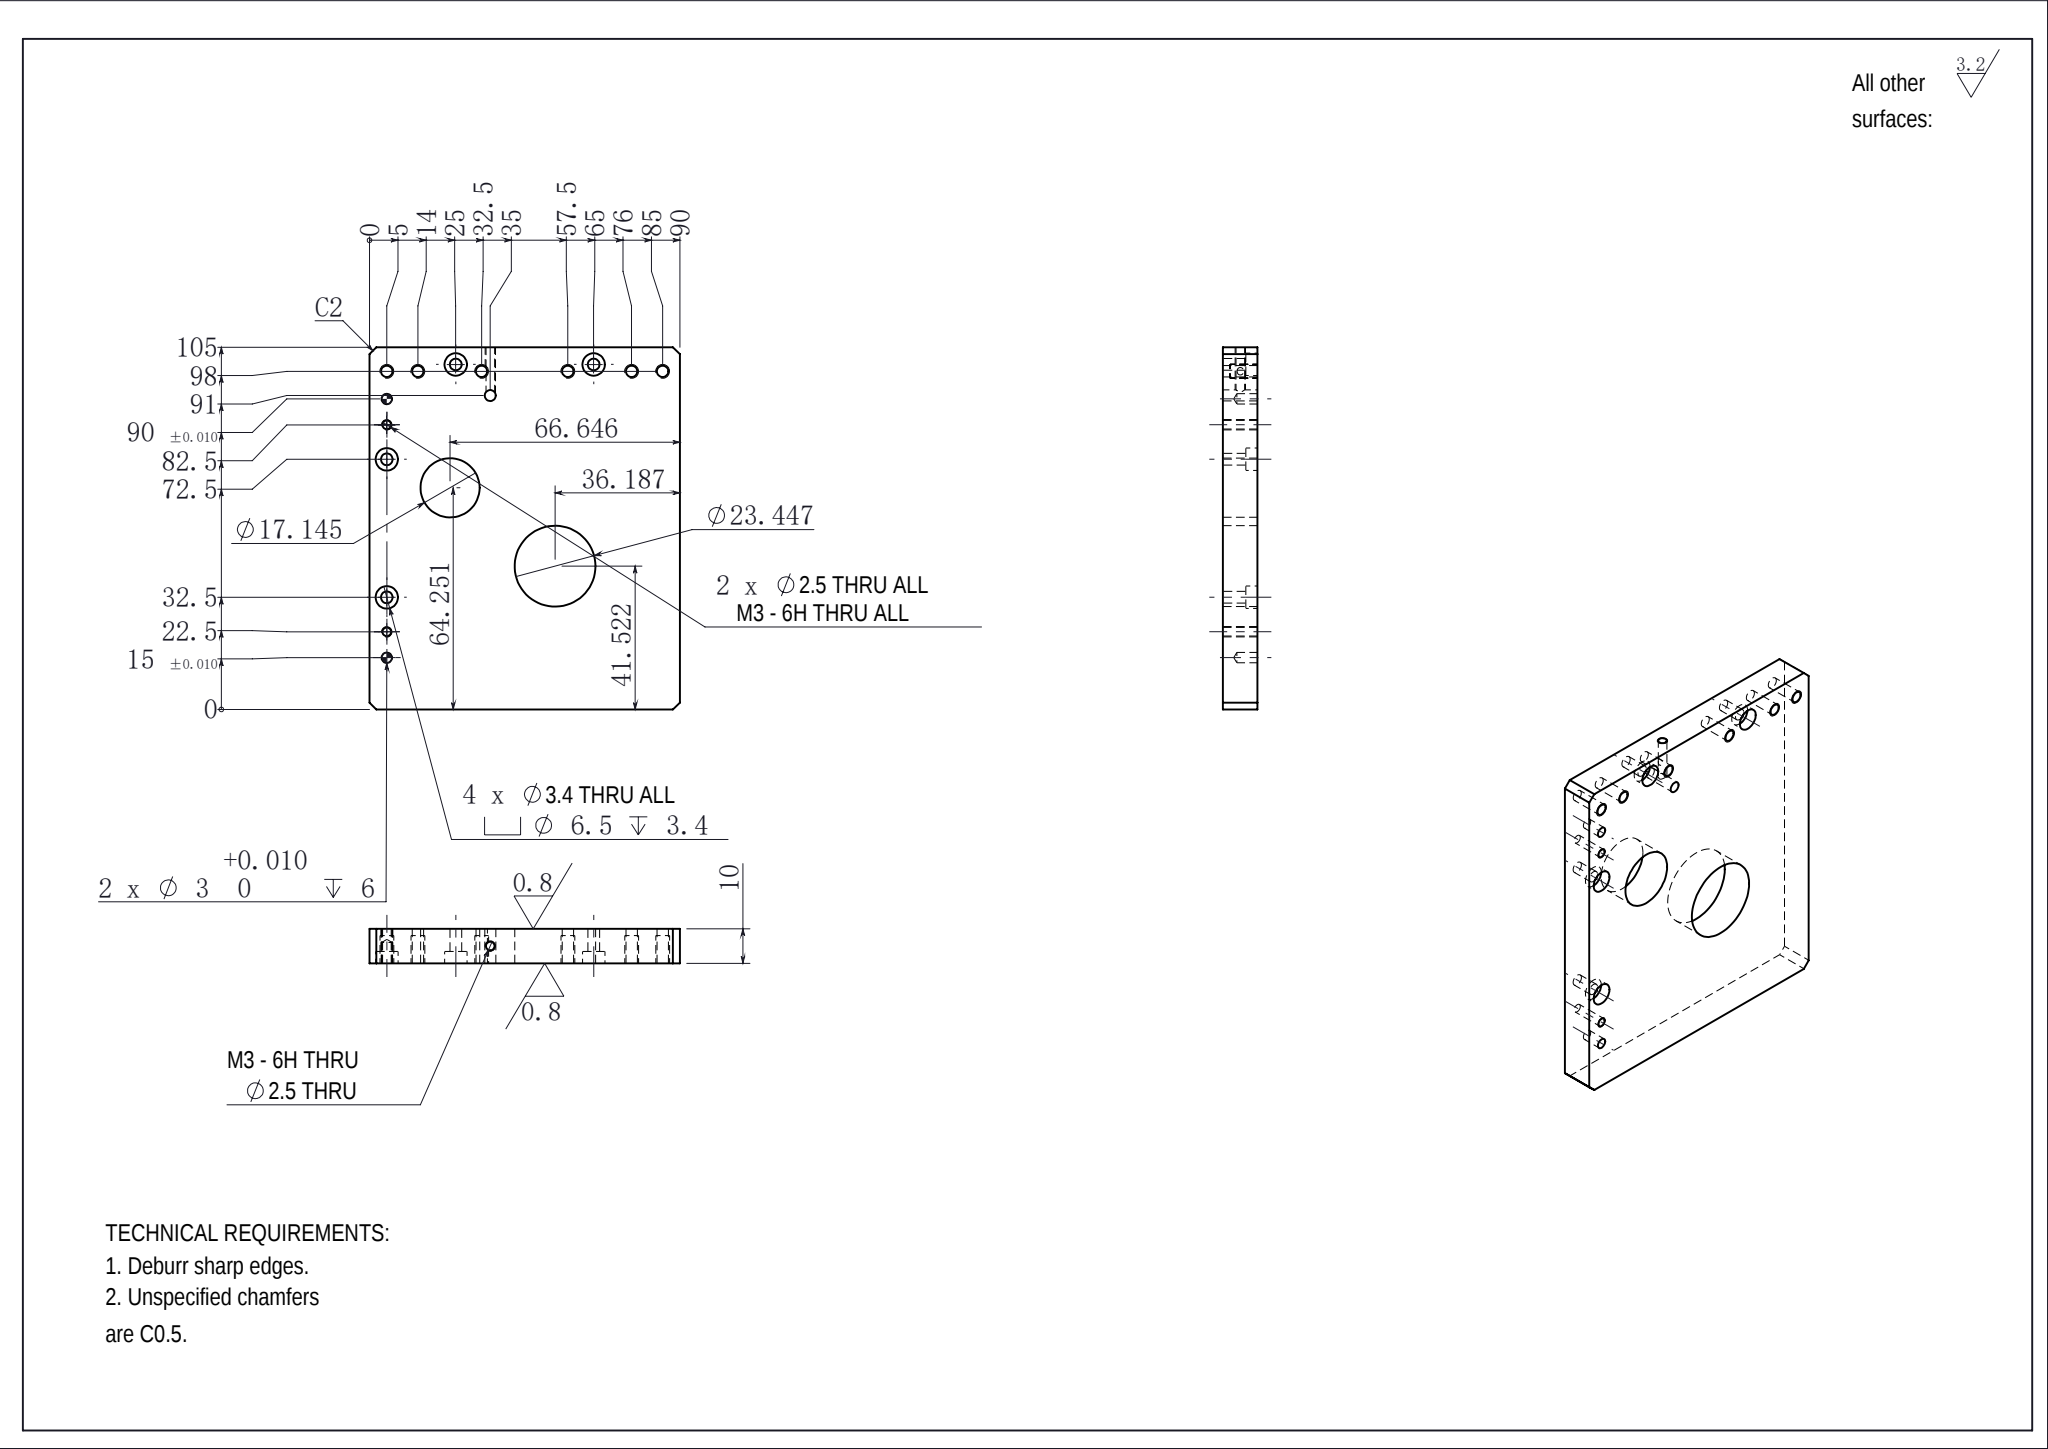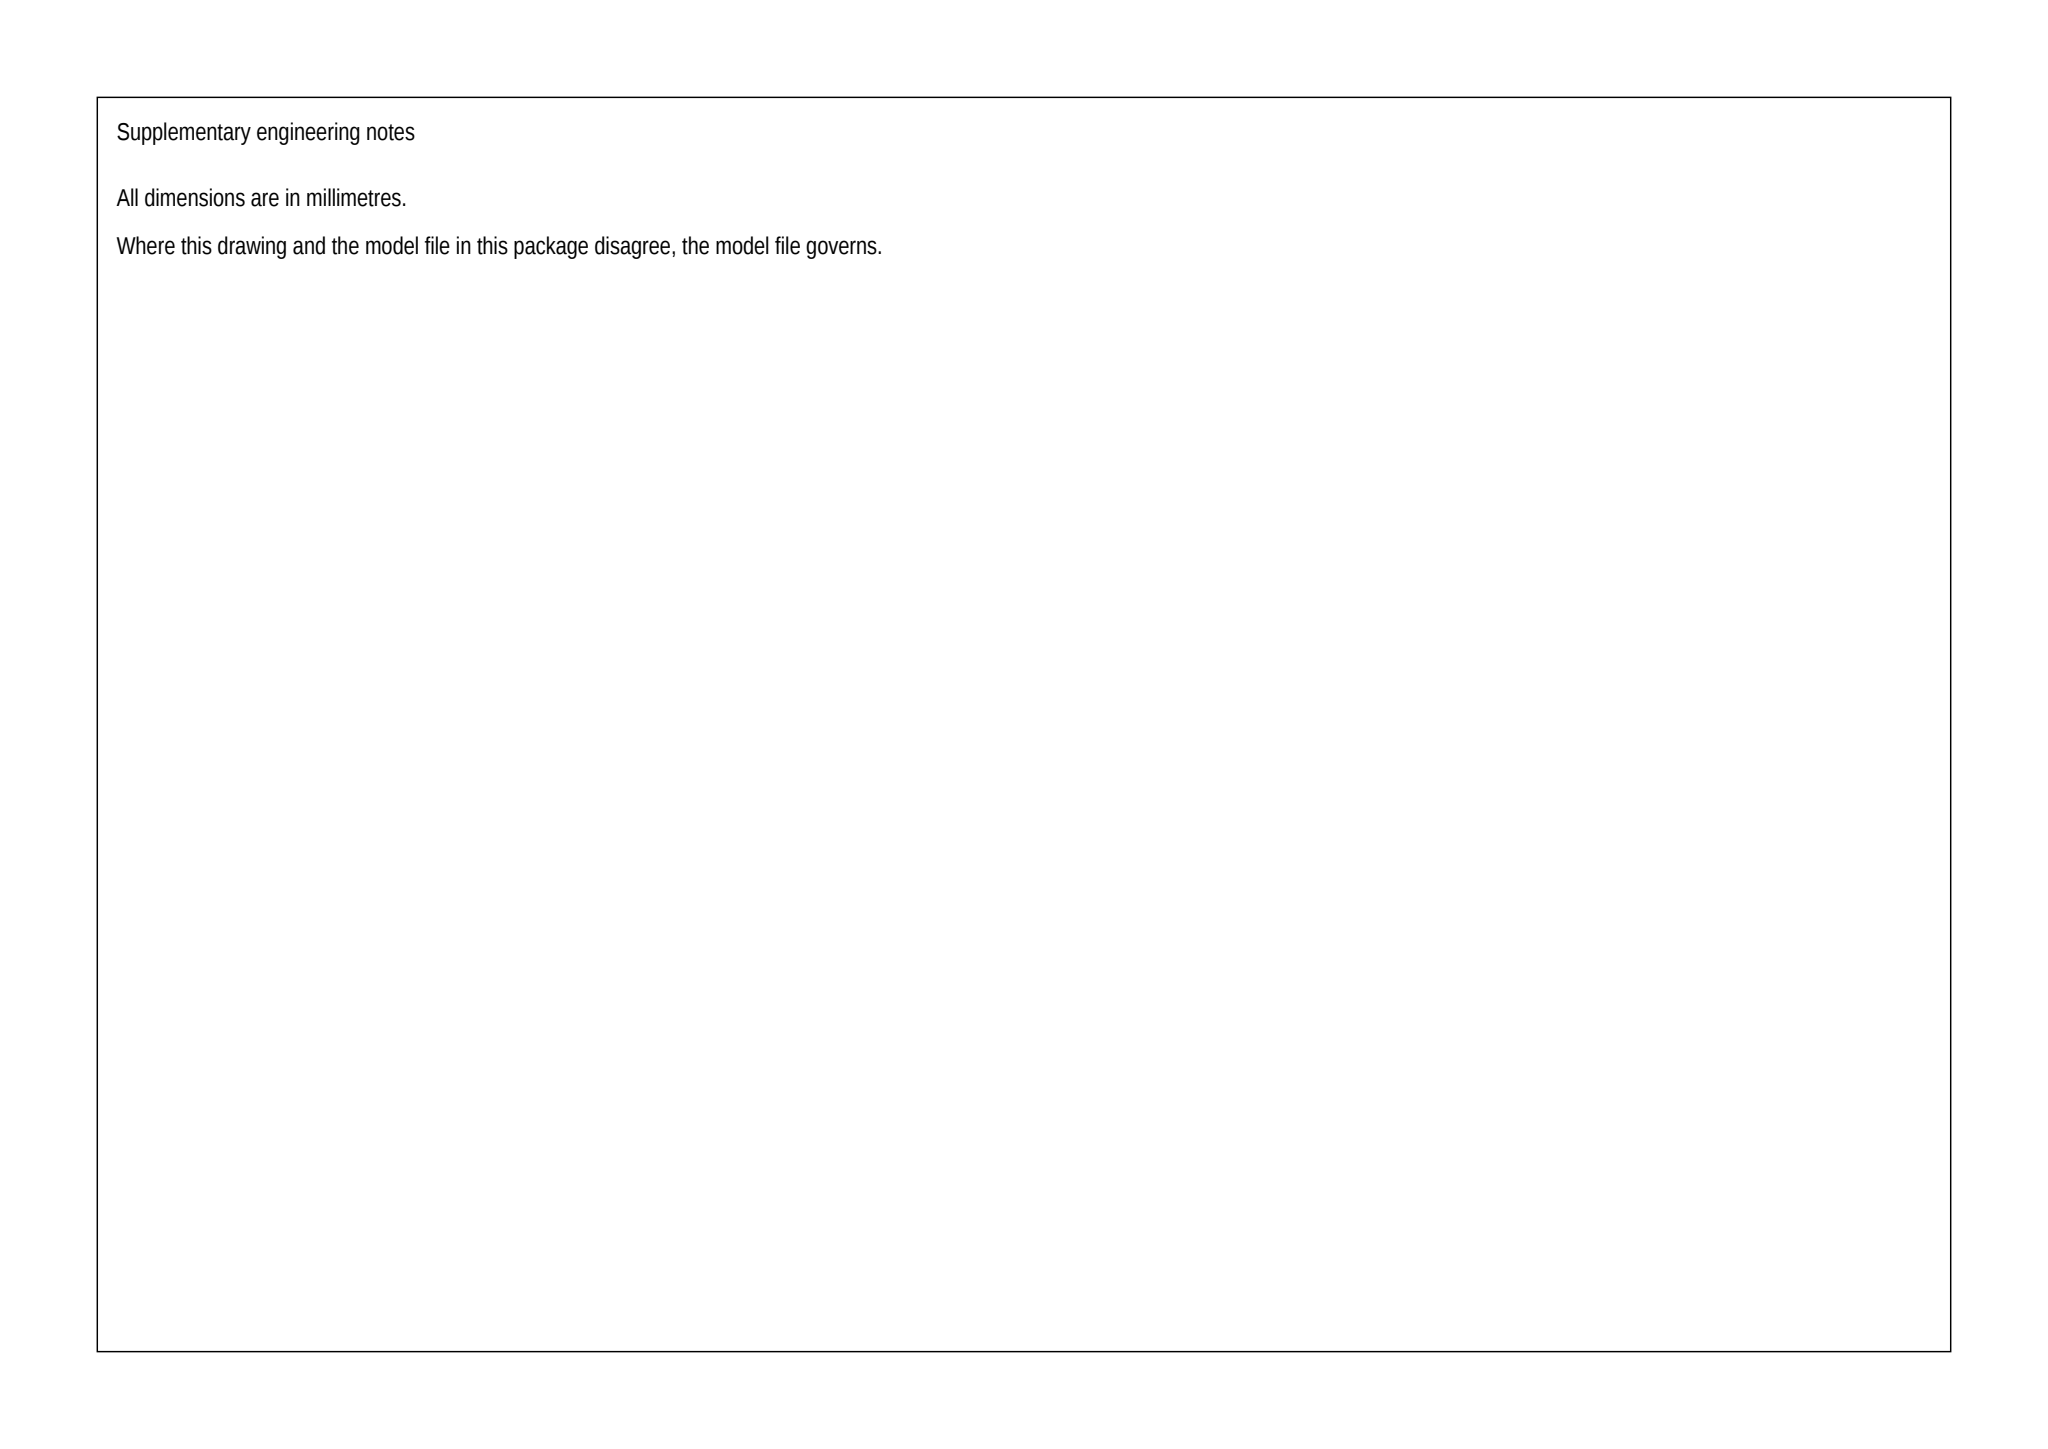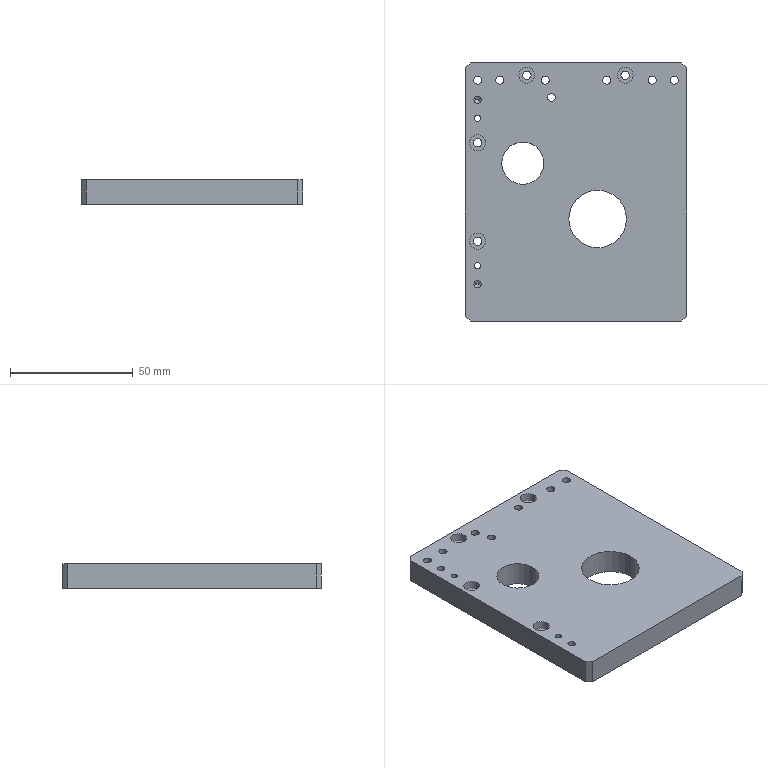Part | SolidWorks | mm | 1 solid | 62 faces | box 90 x 105 x 10 mm | volume 86261 mm3 | cylinder 44 | plane 14 | cone 4 | commonest cylinder face diameters 3.3 x12 6.5 x8 3.4 x8 2.5 x6 3 x4 23.447 x2 17.145 x2 3.2 x2
build123d program:
from build123d import *

# Parameters (mm, degrees)
SKETCH1_W                                       = 90
SKETCH1_H                                       = 105
BOSS_EXTRUDE1_DEPTH                             = 5
M3_HEX_SOCKET_HEAD_CAP_SCREW_CBORE1_D           = 3.4
M3_HEX_SOCKET_HEAD_CAP_SCREW_CBORE1_CBORE_D     = 6.5
M3_HEX_SOCKET_HEAD_CAP_SCREW_CBORE1_CBORE_DEPTH = 3.4
CHAMFER1_SIZE                                   = 2
M3_TAPPED_HOLE1_D                               = 2.5
SIZE_MM_DOWEL_PIN_HOLE_2_D                      = 3
SIZE_MM_DOWEL_PIN_HOLE_2_DEPTH                  = 6
SIZE_MM_DOWEL_PIN_HOLE_2_TIP                    = 0.9013
F_3_2_3_2_DIAMETER_HOLE1_D                      = 3.2
M3_TAPPED_HOLE2_REACH                           = 116.346
M3_TAPPED_HOLE2_BORE_R                          = 1.25
M4_TAPPED_HOLE1_D                               = 3.3
M4_TAPPED_HOLE1_DEPTH                           = 10.1
M4_TAPPED_HOLE1_TIP                             = 0.9914
SKETCH19_R                                      = 11.723
SKETCH19_R_2                                    = 8.573
CUT_EXTRUDE1_DEPTH                              = 80


with BuildPart() as part:
    # Sketch1 → Boss-Extrude1 (new, symmetric)
    with BuildSketch(Plane.XY):
        Rectangle(SKETCH1_W, SKETCH1_H)
    extrude(amount=BOSS_EXTRUDE1_DEPTH, both=True)

    # M3 Hex Socket Head Cap Screw CBORE1 (through all)
    with Locations(Plane.XY.offset(5)):
        with Locations((-40, -20), (-40, 20), (-20, 47.5), (20, 47.5)):
            CounterBoreHole(M3_HEX_SOCKET_HEAD_CAP_SCREW_CBORE1_D / 2, M3_HEX_SOCKET_HEAD_CAP_SCREW_CBORE1_CBORE_D / 2, M3_HEX_SOCKET_HEAD_CAP_SCREW_CBORE1_CBORE_DEPTH)

    # Chamfer1
    chamfer1_edges = [part.edges().sort_by_distance(p)[0] for p in [
        (45, -52.5, 0),
        (-45, -52.5, 0),
        (-45, 52.5, 0),
        (45, 52.5, 0),
    ]]
    chamfer(chamfer1_edges, length=CHAMFER1_SIZE)

    # M3 Tapped Hole1 (through all)
    with Locations(Plane.XY.offset(5)):
        with Locations((-40, 30), (-40, -30)):
            Hole(M3_TAPPED_HOLE1_D / 2)

    # Size mm Dowel Pin Hole 2
    with Locations(Plane.XY.offset(5)):
        with Locations((-40, 37.5), (-40, -37.5)):
            Hole(SIZE_MM_DOWEL_PIN_HOLE_2_D / 2, depth=SIZE_MM_DOWEL_PIN_HOLE_2_DEPTH)
            with Locations((0, 0, -(SIZE_MM_DOWEL_PIN_HOLE_2_DEPTH + SIZE_MM_DOWEL_PIN_HOLE_2_TIP / 2))):  # 118° drill point
                Cone(0, SIZE_MM_DOWEL_PIN_HOLE_2_D / 2, SIZE_MM_DOWEL_PIN_HOLE_2_TIP, mode=Mode.SUBTRACT)

    # 3.2 _3.2_ Diameter Hole1 (through all)
    with Locations(Plane.XY.offset(5)):
        with Locations((-10, 38.5)):
            Hole(F_3_2_3_2_DIAMETER_HOLE1_D / 2)

    # M3 Tapped Hole2 bore → M3 Tapped Hole2 (cut, up to next)
    with BuildSketch(Plane(origin=(0, 52.5, 0), x_dir=(1, 0, 0), z_dir=(0, 1, 0)), mode=Mode.PRIVATE) as m3_tapped_hole2_sk1:
        with Locations((-10, 0)):
            Circle(M3_TAPPED_HOLE2_BORE_R)
    m3_tapped_hole2_tool1 = extrude(m3_tapped_hole2_sk1.sketch, amount=-M3_TAPPED_HOLE2_REACH, mode=Mode.PRIVATE) & part.part
    add(m3_tapped_hole2_tool1.solids().sort_by_distance((-10, 52.5, 0))[0], mode=Mode.SUBTRACT)

    # M4 Tapped Hole1
    with Locations(Plane.XY.offset(5)):
        with Locations((-40, 45.5), (-31, 45.5), (-12.5, 45.5), (12.5, 45.5), (31, 45.5), (40, 45.5)):
            Hole(M4_TAPPED_HOLE1_D / 2, depth=M4_TAPPED_HOLE1_DEPTH)
            with Locations((0, 0, -(M4_TAPPED_HOLE1_DEPTH + M4_TAPPED_HOLE1_TIP / 2))):  # 118° drill point
                Cone(0, M4_TAPPED_HOLE1_D / 2, M4_TAPPED_HOLE1_TIP, mode=Mode.SUBTRACT)

    # Sketch19 → Cut-Extrude1 (cut)
    with BuildSketch(Plane.XY.offset(5)):
        with Locations((8.813, -10.978)):
            Circle(SKETCH19_R)
        with Locations((-21.646, 11.751)):
            Circle(SKETCH19_R_2)
    extrude(amount=-CUT_EXTRUDE1_DEPTH, mode=Mode.SUBTRACT)


solid = part.part